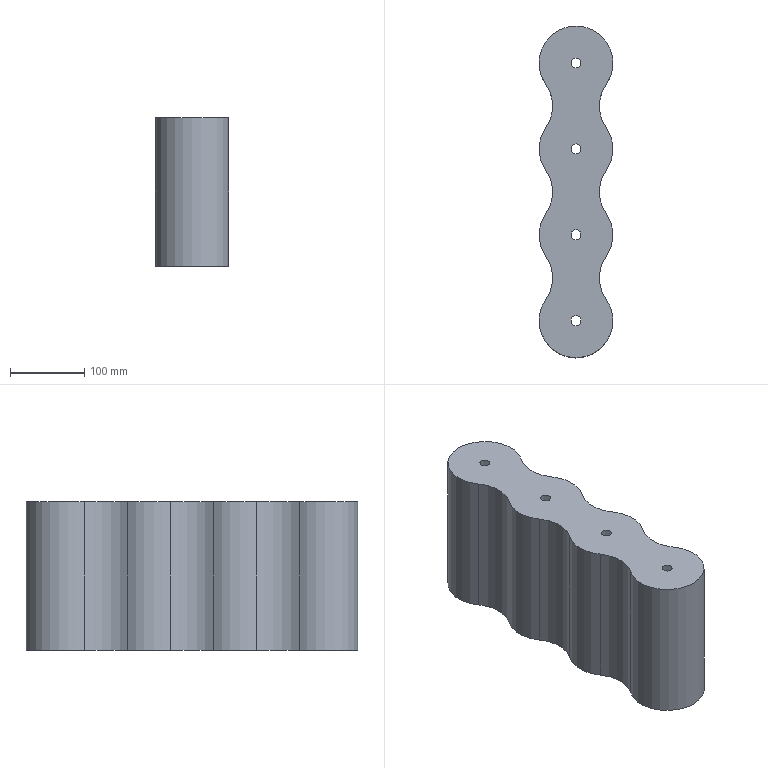Component | NX | CYLINDER | 1 solid | 22 faces | volume 3461094 mm3 | cylinder 16 | cone 4 | plane 2 | commonest cylinder face diameters 100 x12 80 x4